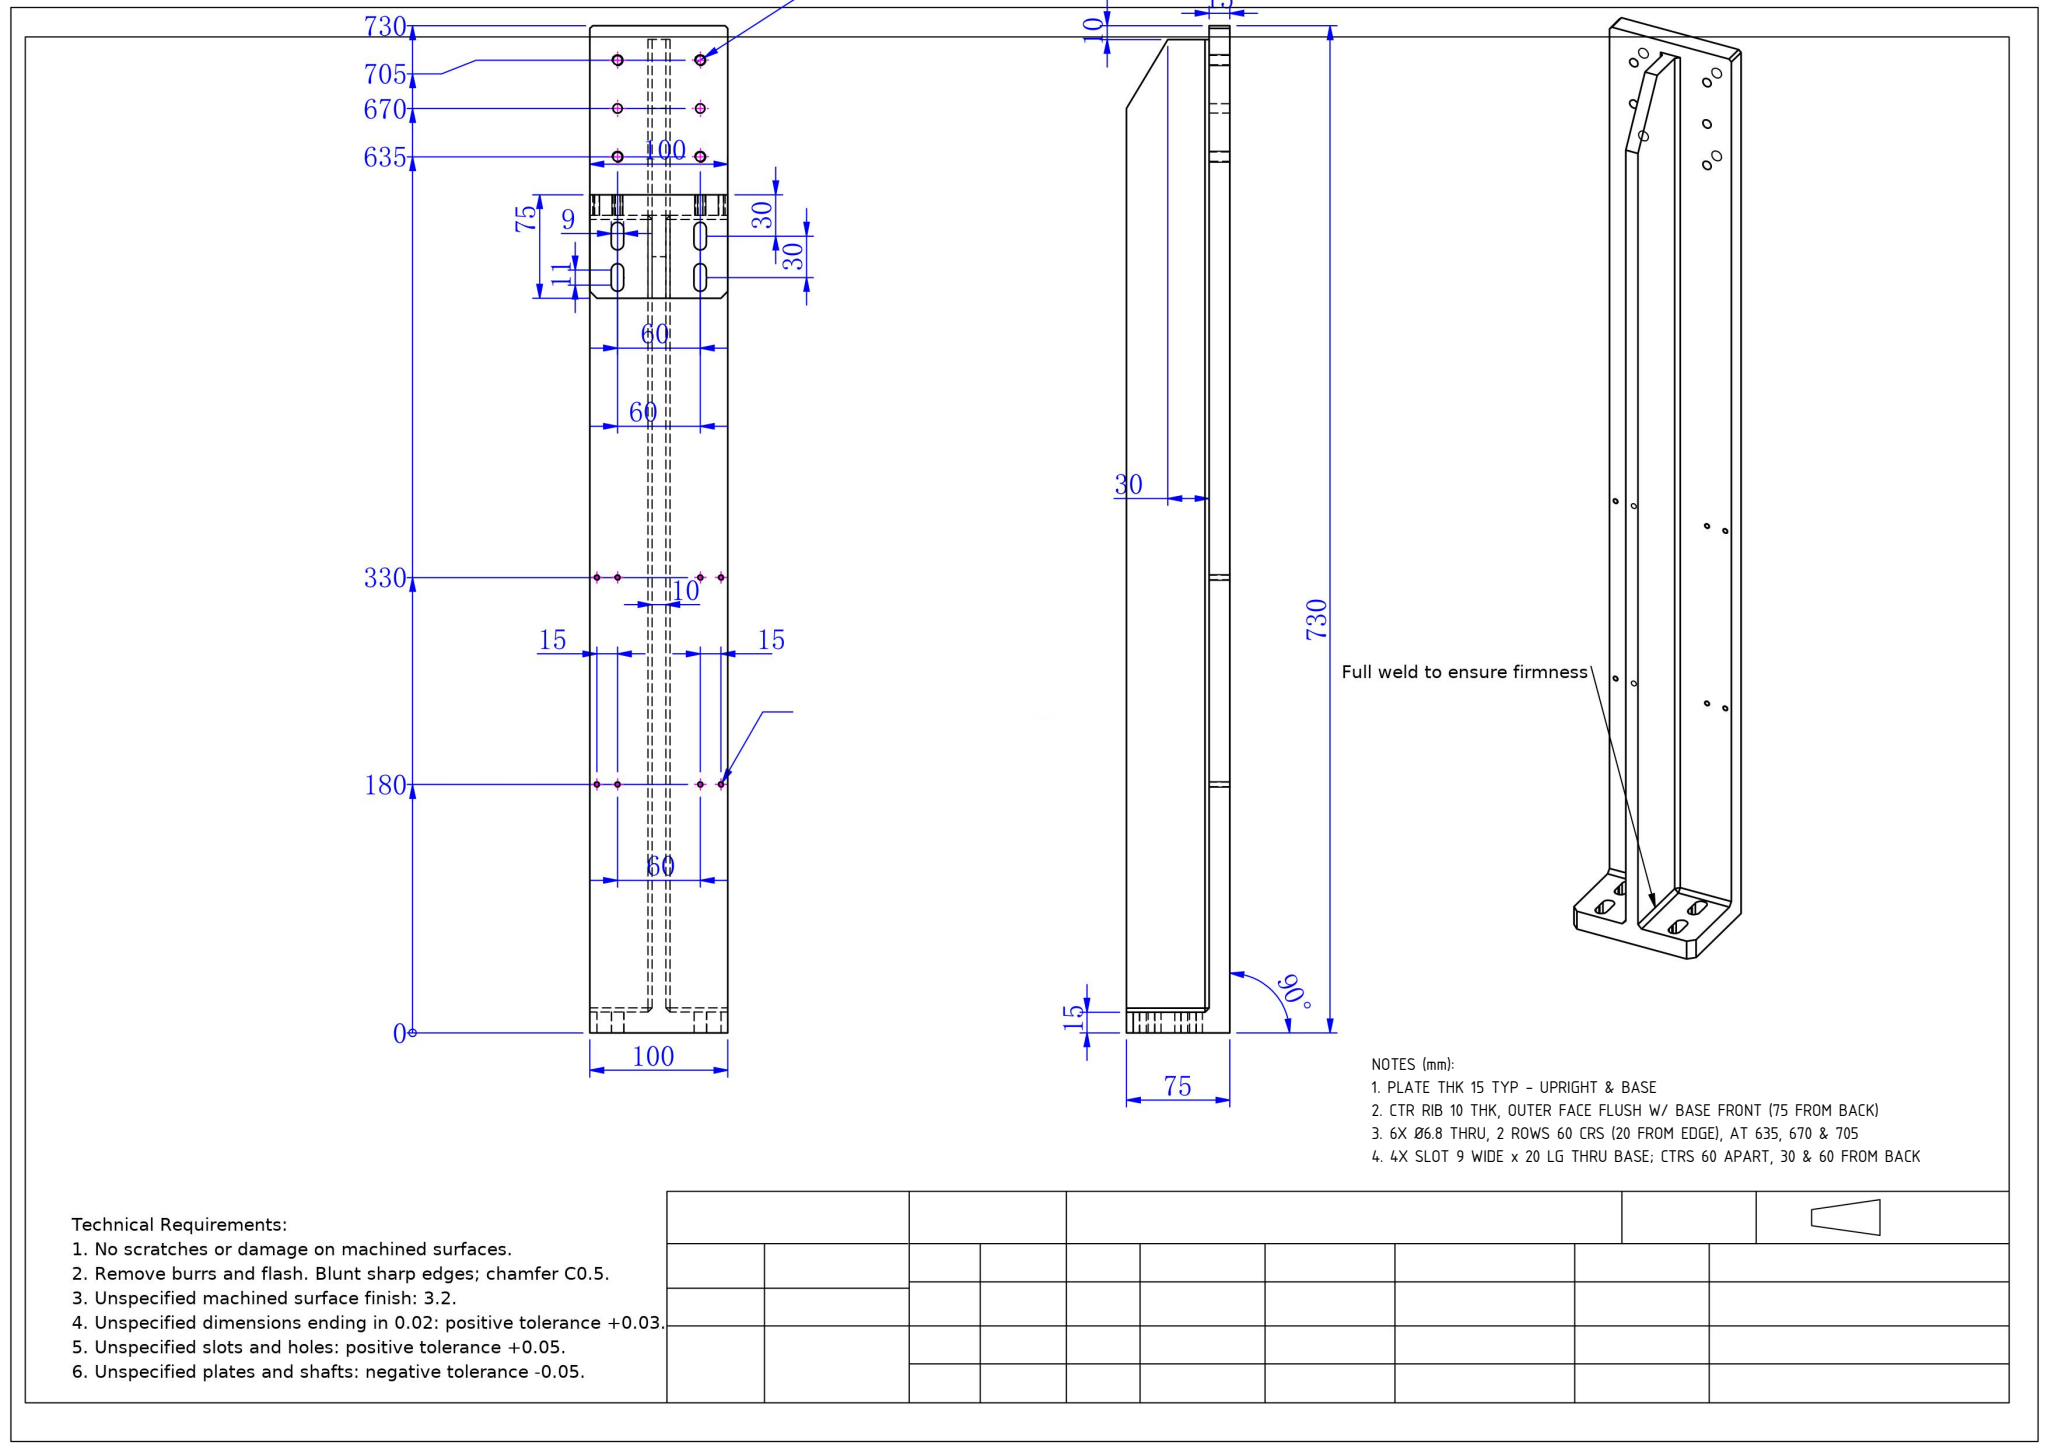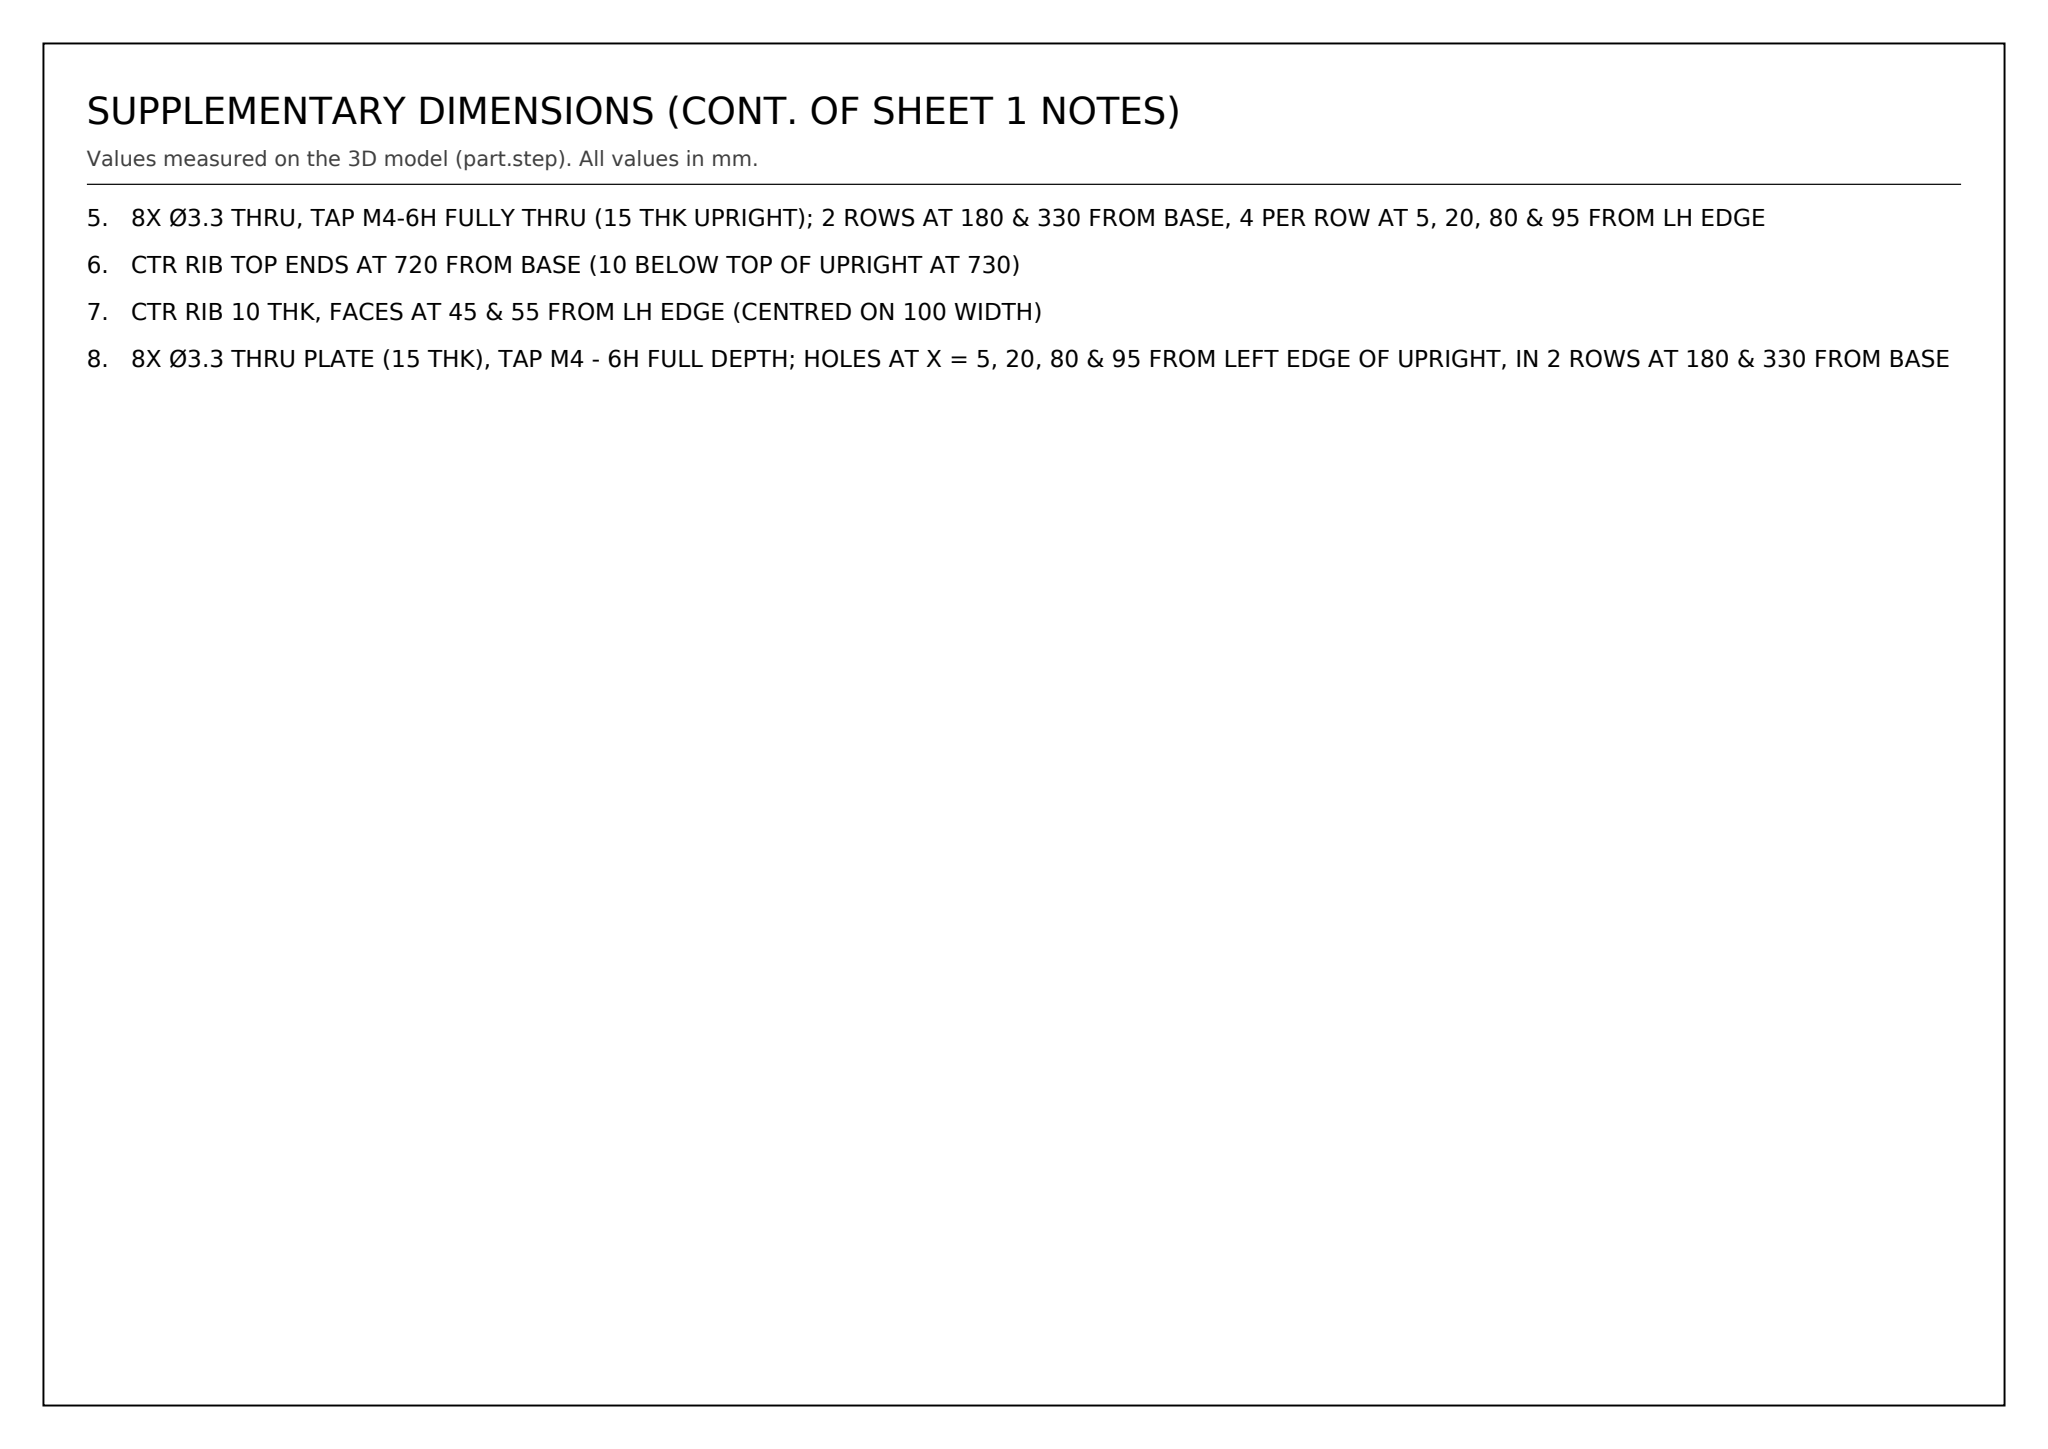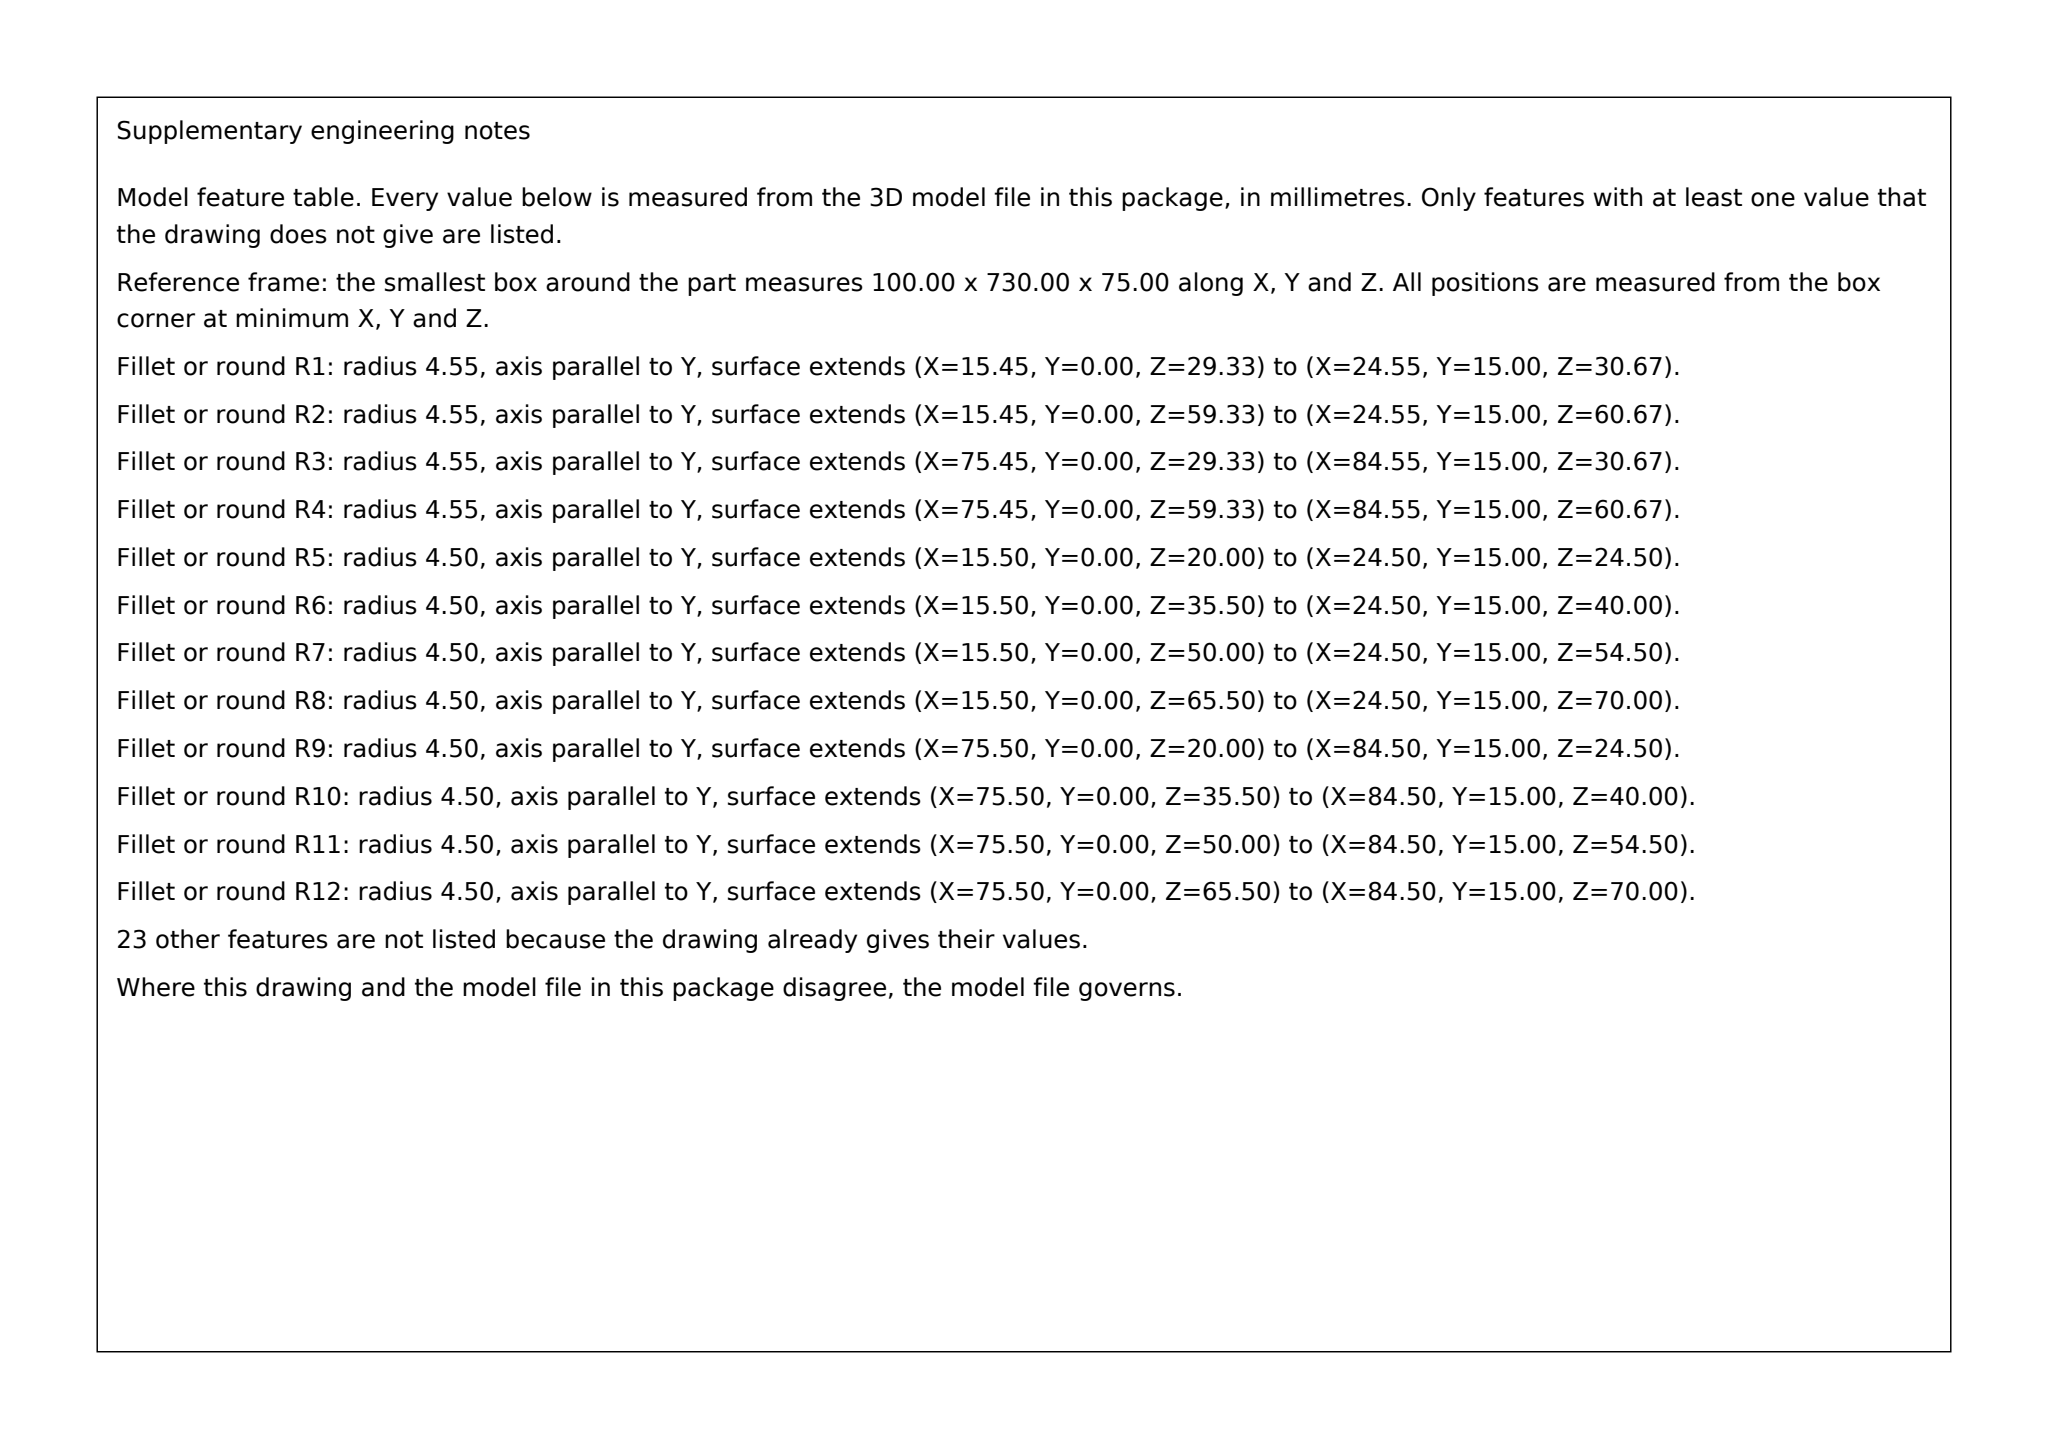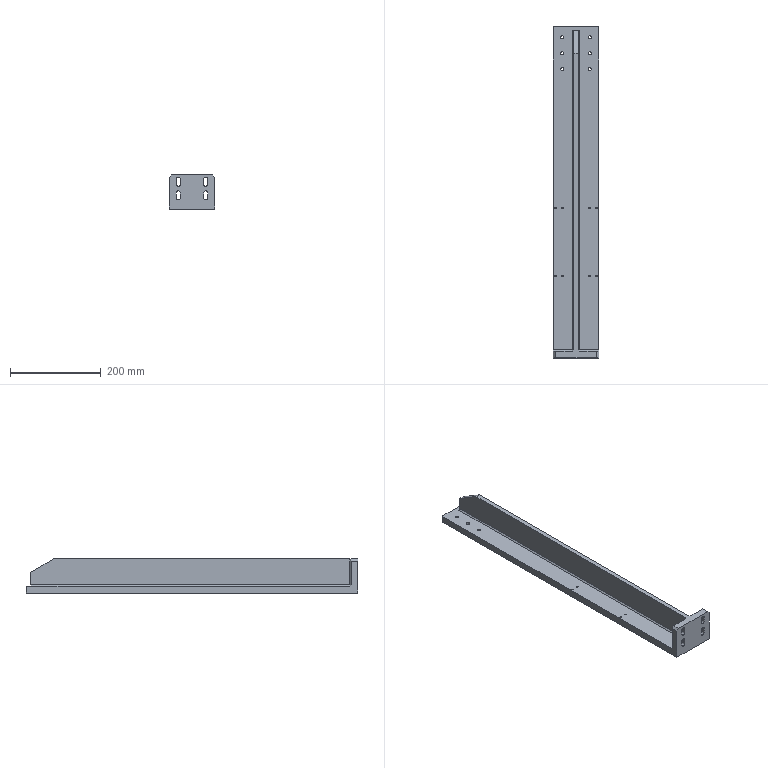Part | SolidWorks | mm | 1 solid | 89 faces | box 100 x 730 x 75 mm | volume 1593262 mm3 | cylinder 48 | plane 41 | commonest cylinder face diameters 3.3 x16 6.8 x12 9 x12 9.1 x8
Drawing notes:
PLATE THK 15 TYP - UPRIGHT & BASE | from the solid: z-planes 0/15 (upright), y-planes 0/15 (base); all thru holes 15 deep
CTR RIB 10 THK, OUTER FACE FLUSH W/ BASE FRONT (75 FROM BACK) | from the solid: x-planes 45 & 55, 10 apart centred on 100 width; z-plane 75 shared with base front
6X Ø6.8 THRU, 2 ROWS 60 CRS (20 FROM EDGE), AT 635, 670 & 705 | from the solid: Ø6.8 z-axis cyls at x=20 & 80, y=635/670/705, length 15 thru plate
4X SLOT 9 WIDE x 20 LG THRU BASE; CTRS 60 APART, 30 & 60 FROM BACK | from the solid: Ø9 y-axis cyls at x=20 & 80, z=24.5/35.5 & 54.5/65.5 (11 crs, 20 OA), 15 thru base
8X Ø3.3 THRU, TAP M4-6H FULLY THRU (15 THK UPRIGHT); 2 ROWS AT 180 & 330 FROM BASE, 4 PER ROW AT 5, 20, 80 & 95 FROM LH EDGE | from the solid: cylinders dia 3.3, axis z, length 15 at x=5,20,80,95 with y=180 and y=330
CTR RIB TOP ENDS AT 720 FROM BASE (10 BELOW TOP OF UPRIGHT AT 730) | from the solid: axis_planes y=720.0 (vs y=730.0 top face)
CTR RIB 10 THK, FACES AT 45 & 55 FROM LH EDGE (CENTRED ON 100 WIDTH) | from the solid: axis_planes x=45.0 and x=55.0 with bbox_xyz x=100.0
8X Ø3.3 THRU PLATE (15 THK), TAP M4 - 6H FULL DEPTH; HOLES AT X = 5, 20, 80 & 95 FROM LEFT EDGE OF UPRIGHT, IN 2 ROWS AT 180 & 330 FROM BASE | from the solid: cylinders dia 3.3, axis z, length 15, positions (5,180),(20,180),(80,180),(95,180),(5,330),(20,330),(80,330),(95,330)